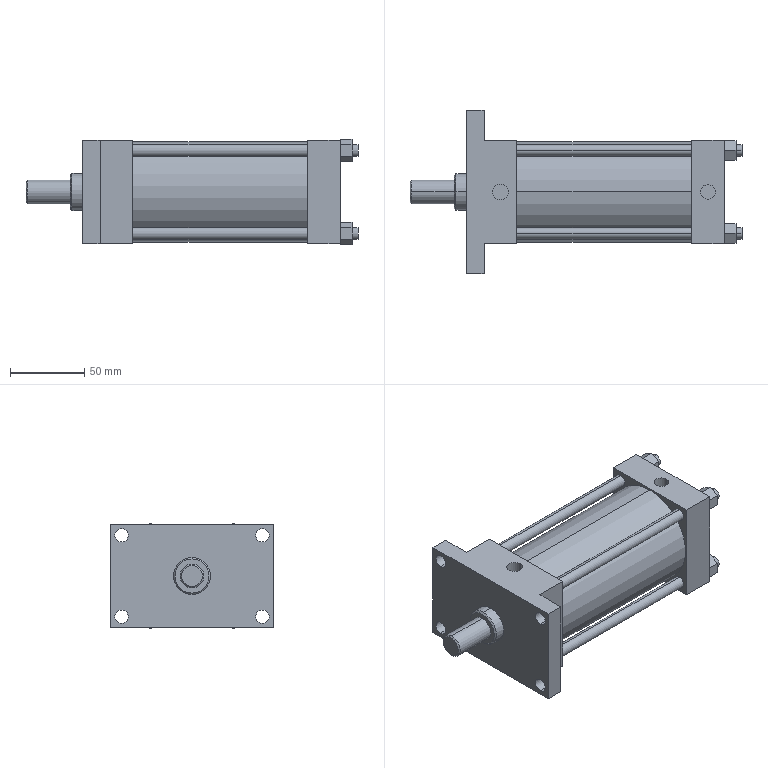Component | SolidWorks | FeedingClampingCylinder-1 | 1 solid | 98 faces | box 224 x 110 x 71.01 mm | volume 535949 mm3 | plane 58 | cylinder 36 | cone 4 | commonest cylinder face diameters 8 x16 9 x8 25 x2 16 x2 9.892 x2 10.599 x2 68 x2 50 x2
build123d program:
from build123d import *

# Parameters (mm, degrees)
SKETCH1_W           = 70
SKETCH1_H           = 70
BOSS_EXTRUDE1_DEPTH = 22
SKETCH2_R           = 34
SKETCH2_R_2         = 25
BOSS_EXTRUDE2_DEPTH = 118
SKETCH3_W           = 70
SKETCH3_H           = 70
BOSS_EXTRUDE3_DEPTH = 22
SKETCH4_R           = 12.5
BOSS_EXTRUDE4_DEPTH = 20
SKETCH5_R           = 8
BOSS_EXTRUDE5_DEPTH = 30
SKETCH7_R           = 5.3
SKETCH7_R_2         = 4.946
CUT_EXTRUDE2_DEPTH  = 30
SKETCH8_R           = 4
BOSS_EXTRUDE6_DEPTH = 152
CHAMFER1_SIZE       = 1
SKETCH9_W           = 70
SKETCH9_H           = 110
SKETCH9_R           = 4.5
BOSS_EXTRUDE7_DEPTH = 12
BOSS_EXTRUDE8_START = 12
SKETCH10_R          = 4
BOSS_EXTRUDE8_DEPTH = 12
BOSS_EXTRUDE9_DEPTH = 8


with BuildPart() as part:
    # Sketch1 → Boss-Extrude1 (new body)
    with BuildSketch(Plane.XY):
        with Locations((35, -35)):
            Rectangle(SKETCH1_W, SKETCH1_H)
    extrude(amount=BOSS_EXTRUDE1_DEPTH)

    # Sketch2 → Boss-Extrude2 (add)
    with BuildSketch(Plane.XY.offset(22)):
        with Locations((35, -35)):
            Circle(SKETCH2_R)
        with Locations((35, -35)):
            Circle(SKETCH2_R_2, mode=Mode.SUBTRACT)
    extrude(amount=BOSS_EXTRUDE2_DEPTH)

    # Sketch3 → Boss-Extrude3 (add)
    with BuildSketch(Plane.XY.offset(140)):
        with Locations((35, -35)):
            Rectangle(SKETCH3_W, SKETCH3_H)
    extrude(amount=BOSS_EXTRUDE3_DEPTH)

    # Sketch4 → Boss-Extrude4 (add)
    with BuildSketch(Plane.XY.offset(162)):
        with Locations((35, -35)):
            Circle(SKETCH4_R)
    extrude(amount=BOSS_EXTRUDE4_DEPTH)

    # Sketch5 → Boss-Extrude5 (add)
    with BuildSketch(Plane.XY.offset(182)):
        with Locations((35, -35)):
            Circle(SKETCH5_R)
    extrude(amount=BOSS_EXTRUDE5_DEPTH)

    # Sketch7 → Cut-Extrude2 (cut)
    with BuildSketch(Plane(origin=(70, 0, 0), x_dir=(0, 0, -1), z_dir=(1, 0, 0))):
        with Locations((-151, -35)):
            Circle(SKETCH7_R)
        with Locations((-11, -35)):
            Circle(SKETCH7_R_2)
    extrude(amount=-CUT_EXTRUDE2_DEPTH, mode=Mode.SUBTRACT)

    # Sketch8 → Boss-Extrude6 (add)
    with BuildSketch(Plane.XY.offset(22)):
        with Locations((7, -7)):
            Circle(SKETCH8_R)
        with Locations((63, -7)):
            Circle(SKETCH8_R)
        with Locations((63, -63)):
            Circle(SKETCH8_R)
        with Locations((7, -63)):
            Circle(SKETCH8_R)
    extrude(amount=BOSS_EXTRUDE6_DEPTH)

    # Chamfer1
    chamfer1_edges = [part.edges().sort_by_distance(p)[0] for p in [
        (22.5, -35, 182),
        (27, -35, 212),
    ]]
    chamfer(chamfer1_edges, length=CHAMFER1_SIZE)

    # Sketch9 → Boss-Extrude7 (add)
    with BuildSketch(Plane.XY.offset(162)):
        with Locations((35, -35)):
            Rectangle(SKETCH9_W, SKETCH9_H)
        with Locations((7.5, 12.5)):
            Circle(SKETCH9_R, mode=Mode.SUBTRACT)
        with Locations((62.5, 12.5)):
            Circle(SKETCH9_R, mode=Mode.SUBTRACT)
        with Locations((7.5, -82.5)):
            Circle(SKETCH9_R, mode=Mode.SUBTRACT)
        with Locations((62.5, -82.5)):
            Circle(SKETCH9_R, mode=Mode.SUBTRACT)
    extrude(amount=BOSS_EXTRUDE7_DEPTH)

    # Sketch10 → Boss-Extrude8 (add)
    with BuildSketch(Plane(origin=(0, 0, 0), x_dir=(-1, 0, 0), z_dir=(0, 0, -1)).offset(BOSS_EXTRUDE8_START)):
        with Locations(Location((-63, -7, 0), (0, 0, 180))):
            Circle(SKETCH10_R)
        with Locations(Location((-7, -7, 0), (0, 0, 180))):
            Circle(SKETCH10_R)
        with Locations(Location((-63, -63, 0), (0, 0, 180))):
            Circle(SKETCH10_R)
        with Locations(Location((-7, -63, 0), (0, 0, 180))):
            Circle(SKETCH10_R)
    extrude(amount=-BOSS_EXTRUDE8_DEPTH)

    # Sketch11 → Boss-Extrude9 (add)
    with BuildSketch(Plane(origin=(0, 0, 0), x_dir=(-1, 0, 0), z_dir=(0, 0, -1))):
        Polygon((-55.494, -7), (-59.247, -0.5), (-66.753, -0.5), (-70.506, -7), (-66.753, -13.5), (-59.247, -13.5), align=None)
        Polygon((0.5056, -7), (-3.247, -0.5), (-10.753, -0.5), (-14.506, -7), (-10.753, -13.5), (-3.247, -13.5), align=None)
        Polygon((-55.494, -63), (-59.247, -56.5), (-66.753, -56.5), (-70.506, -63), (-66.753, -69.5), (-59.247, -69.5), align=None)
        Polygon((0.5056, -63), (-3.247, -56.5), (-10.753, -56.5), (-14.506, -63), (-10.753, -69.5), (-3.247, -69.5), align=None)
    extrude(amount=BOSS_EXTRUDE9_DEPTH)


solid = part.part

# Placed as in the assembly
solid = solid.moved(Location((256.191, 30.819, -35), (0, -90, 0)))